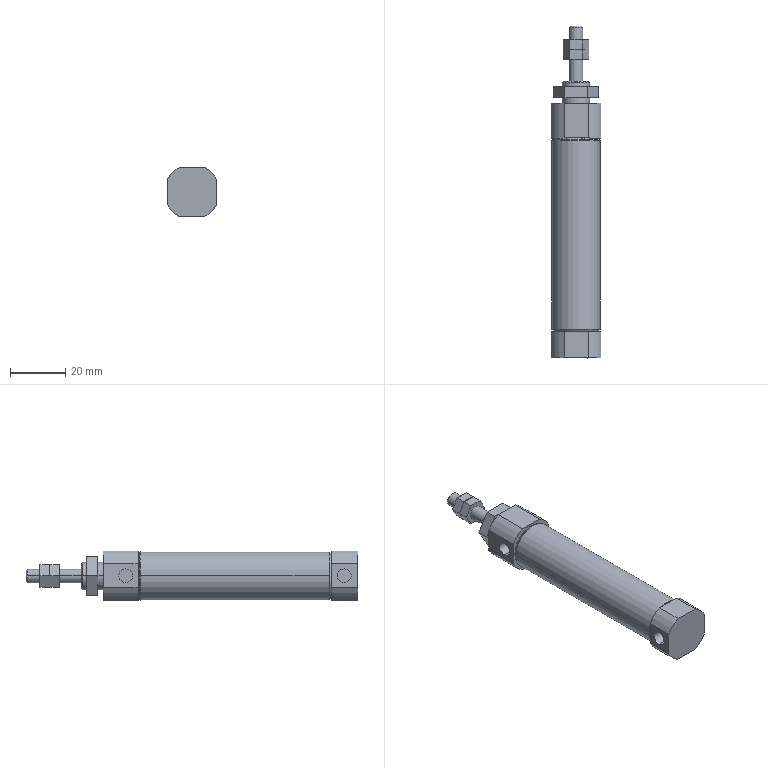Component | SolidWorks | AB16X45-1 | 1 solid | 76 faces | box 18.07 x 120 x 18.07 mm | volume 24454 mm3 | plane 40 | cylinder 24 | cone 8 | spline 4 | commonest cylinder face diameters 5 x10 20 x8 10 x4 17.4 x2